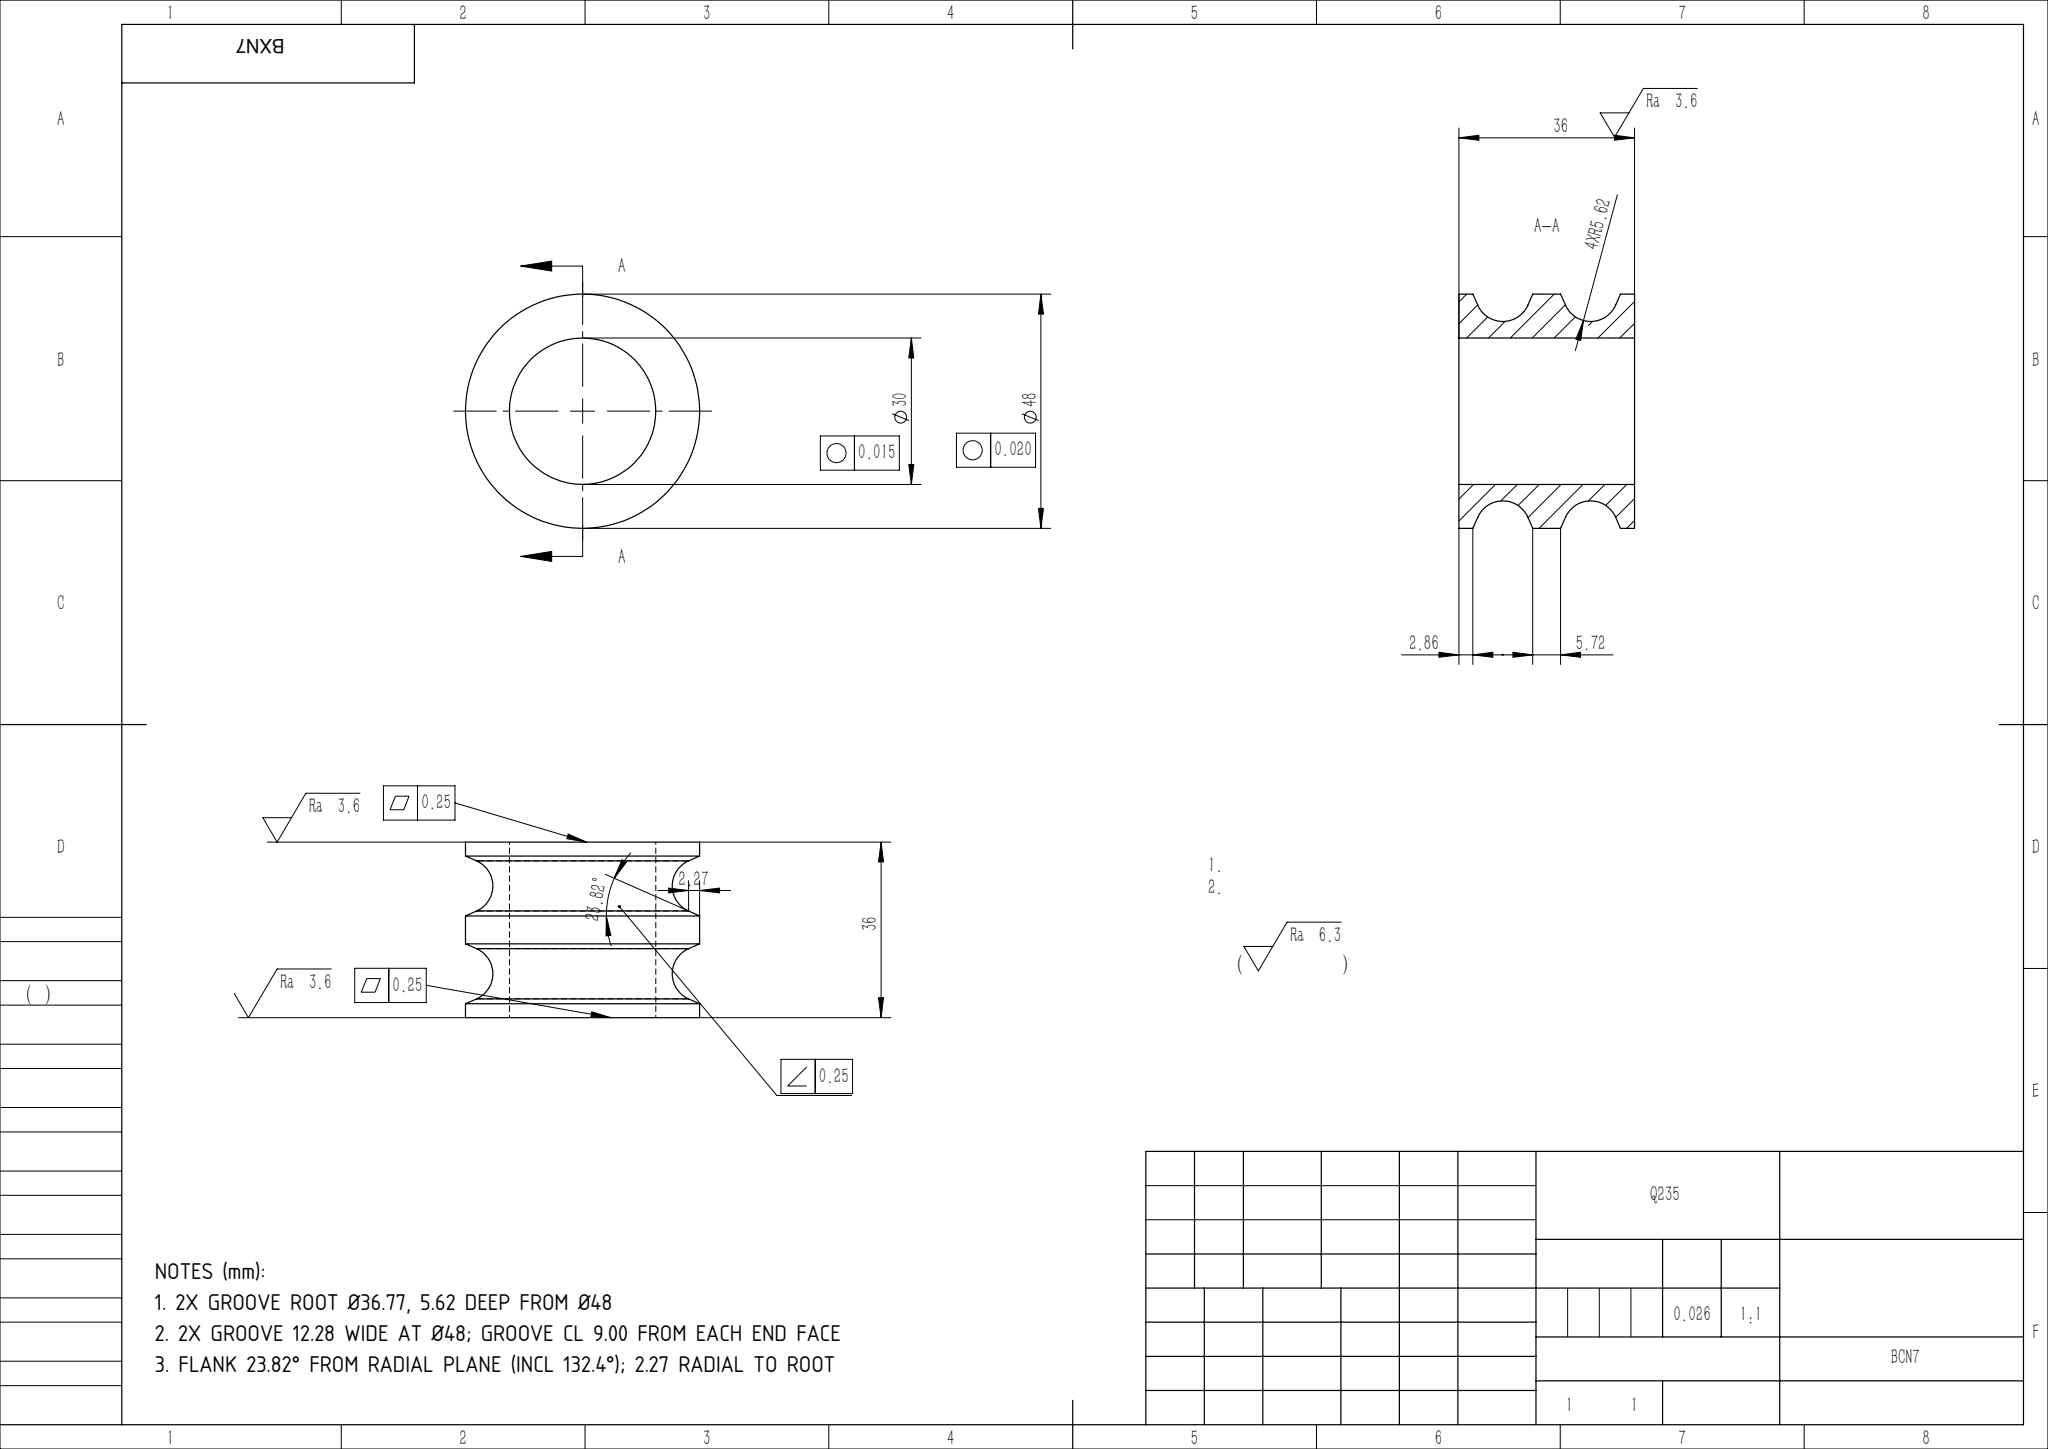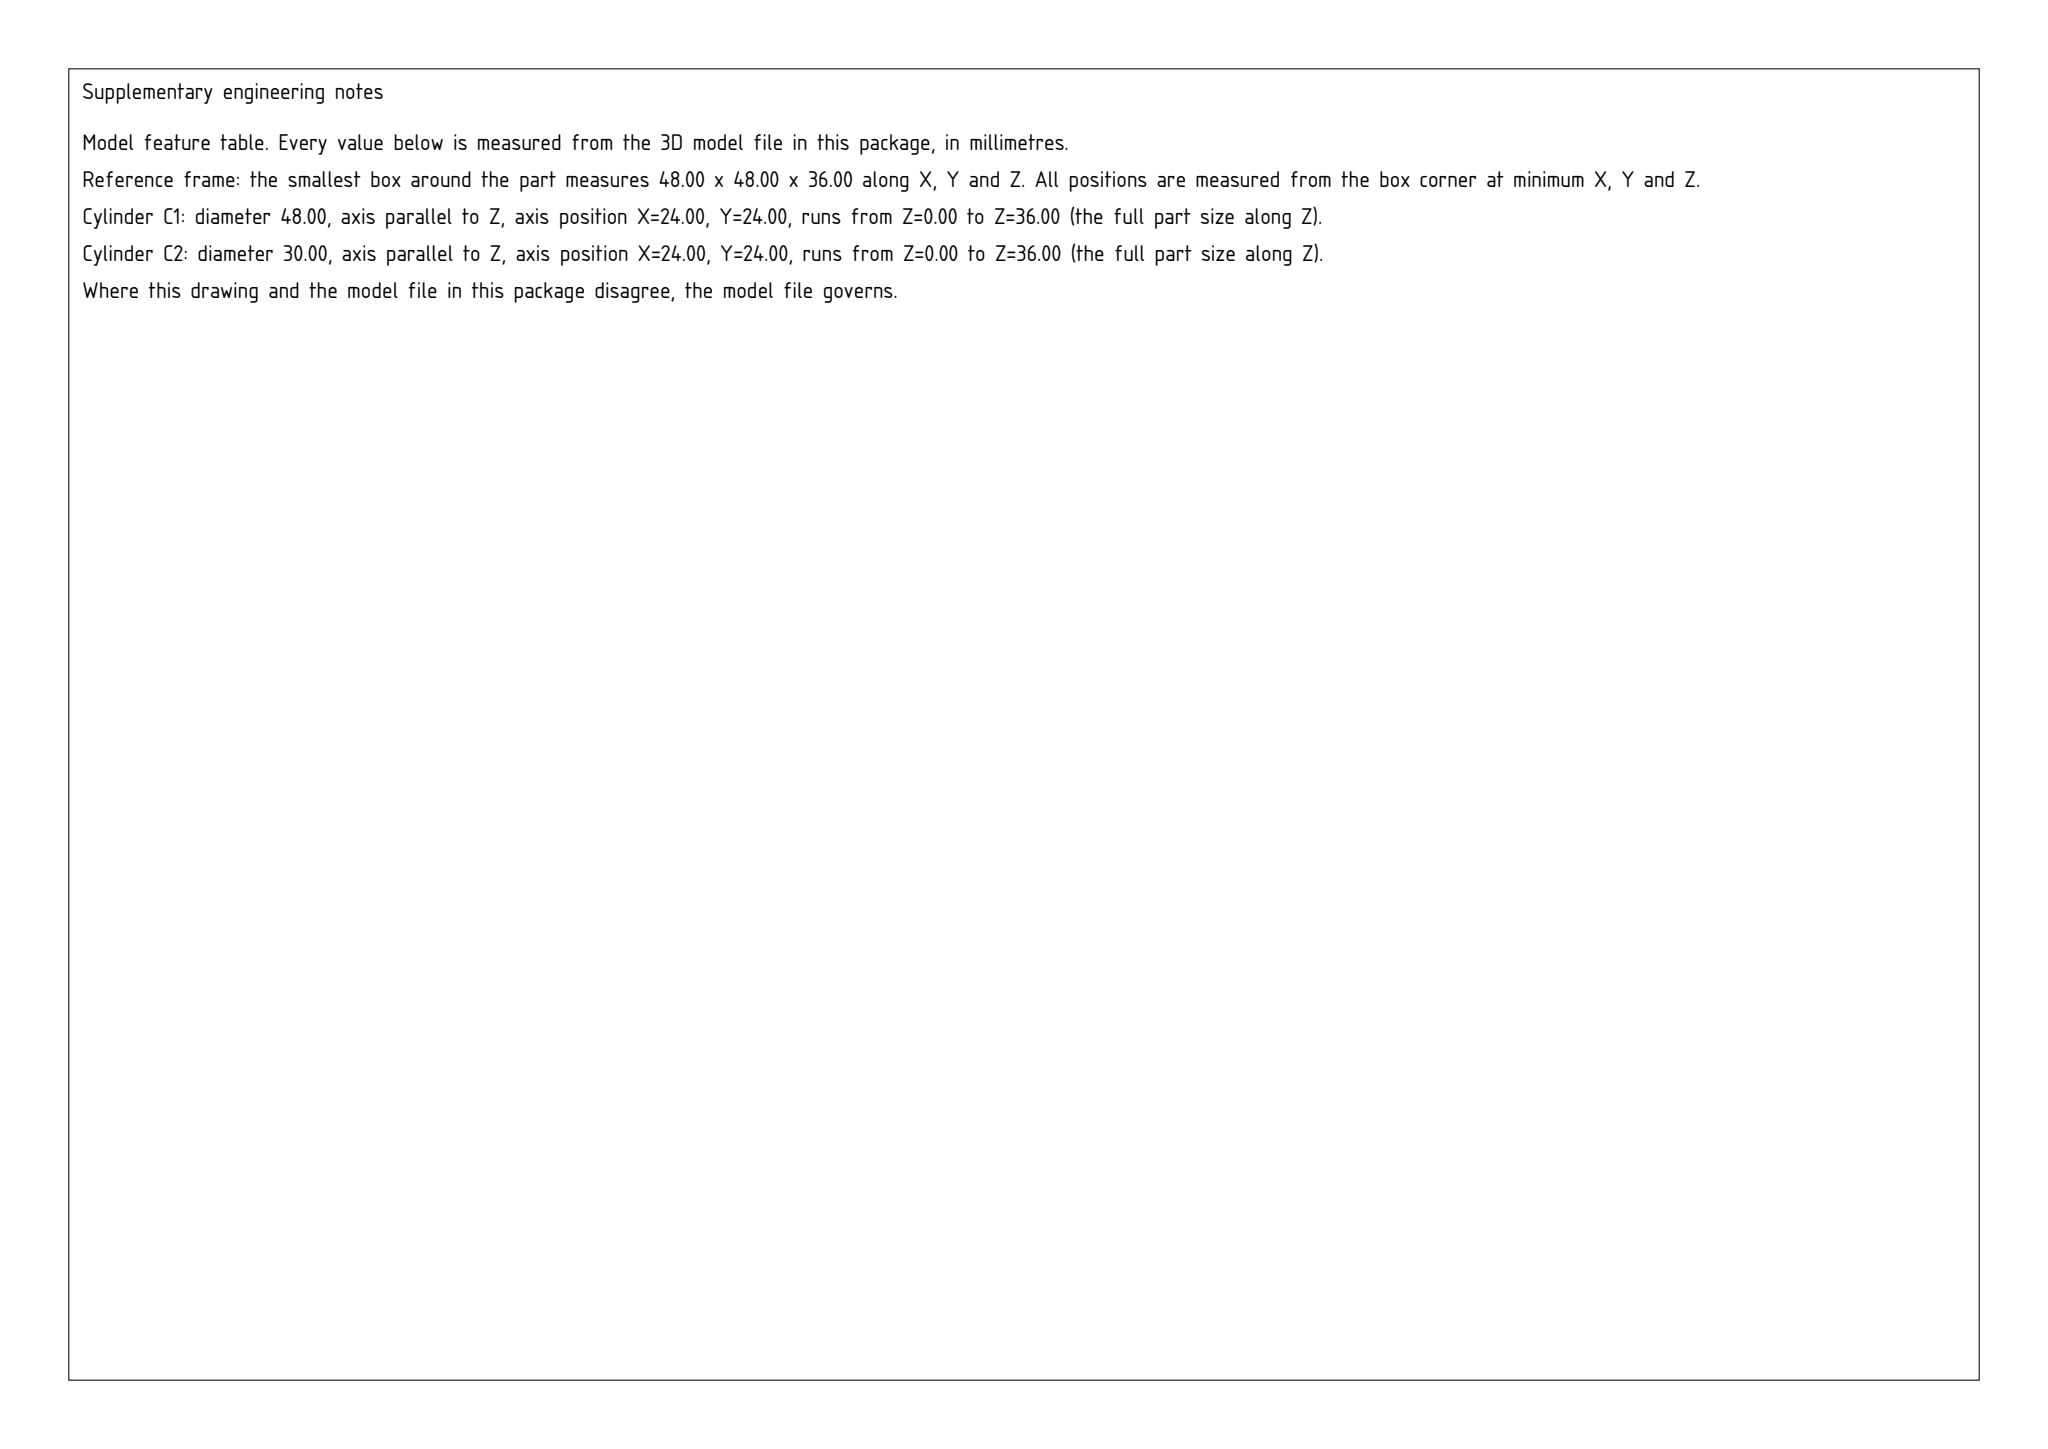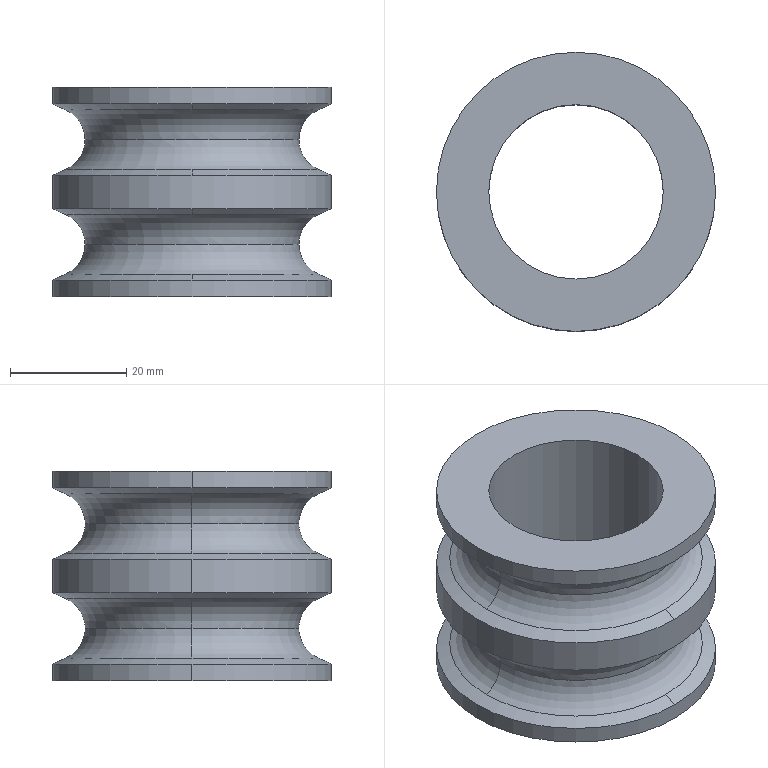Part | SolidWorks | mm | material Q235 | 1 solid | 26 faces | box 48 x 48 x 36 mm | volume 26002 mm3 | torus 8 | cylinder 8 | cone 8 | plane 2 | commonest cylinder face diameters 48 x6 30 x2
Drawing notes:
2X GROOVE ROOT Ø36.77, 5.62 DEEP FROM Ø48 | from the solid: cones incl angle 132.4 ref dia 48 tangent to R5.616 fillets -> root radius 18.384 (24-5.616), depth = R = 5.616
2X GROOVE 12.28 WIDE AT Ø48; GROOVE CL 9.00 FROM EACH END FACE | from the solid: 36 overall - (2.86+5.72+2.86) Ø48 lands = 24.56 / 2 grooves = 12.28 ea; CL = 2.86+6.14 = 9.00 from z=0 and z=36 faces
FLANK 23.82° FROM RADIAL PLANE (INCL 132.4°); 2.27 RADIAL TO ROOT | from the solid: cone included angle 132.4 deg about z = 23.8 deg from plane normal to axis; cone radial extent 20.652->18.384 = 2.268
STEP:
#1=CARTESIAN_POINT('',(-21.732,0.,-14.137));
#2=VERTEX_POINT('',#1);
#3=CARTESIAN_POINT('',(-18.384,0.,-9.));
#4=VERTEX_POINT('',#3);
#5=CARTESIAN_POINT('',(-24.,0.,-9.));
#6=DIRECTION('',(0.,-1.,0.));
#7=DIRECTION('',(0.,0.,-1.));
#8=AXIS2_PLACEMENT_3D('',#5,#6,#7);
#9=CIRCLE('',#8,5.616);
#10=EDGE_CURVE('',#2,#4,#9,.T.);
#11=ORIENTED_EDGE('',*,*,#10,.T.);
#12=CARTESIAN_POINT('',(18.384,0.,-9.));
#13=VERTEX_POINT('',#12);
#14=CARTESIAN_POINT('',(0.,0.,-9.));
#15=DIRECTION('',(0.,0.,-1.));
#16=DIRECTION('',(-1.,0.,0.));
#17=AXIS2_PLACEMENT_3D('',#14,#15,#16);
#18=CIRCLE('',#17,18.384);
#19=EDGE_CURVE('',#4,#13,#18,.T.);
#20=ORIENTED_EDGE('',*,*,#19,.T.);
#21=CARTESIAN_POINT('',(21.732,0.,-14.137));
#22=VERTEX_POINT('',#21);
#23=CARTESIAN_POINT('',(24.,0.,-9.));
#24=DIRECTION('',(-0.,1.,0.));
#25=DIRECTION('',(-1.,-0.,0.));
#26=AXIS2_PLACEMENT_3D('',#23,#24,#25);
#27=CIRCLE('',#26,5.616);
#28=EDGE_CURVE('',#22,#13,#27,.T.);
#29=ORIENTED_EDGE('',*,*,#28,.F.);
#30=CARTESIAN_POINT('',(0.,21.732,-14.137));
#31=VERTEX_POINT('',#30);
#32=CARTESIAN_POINT('',(0.,0.,-14.137));
#33=DIRECTION('',(0.,0.,-1.));
#34=DIRECTION('',(-1.,0.,0.));
#35=AXIS2_PLACEMENT_3D('',#32,#33,#34);
#36=CIRCLE('',#35,21.732);
#37=EDGE_CURVE('',#31,#22,#36,.T.);
#38=ORIENTED_EDGE('',*,*,#37,.F.);
#39=CARTESIAN_POINT('',(0.,0.,-14.137));
#40=DIRECTION('',(0.,0.,-1.));
#41=DIRECTION('',(-1.,0.,0.));
#42=AXIS2_PLACEMENT_3D('',#39,#40,#41);
#43=CIRCLE('',#42,21.732);
#44=EDGE_CURVE('',#2,#31,#43,.T.);
#45=ORIENTED_EDGE('',*,*,#44,.F.);
#46=EDGE_LOOP('',(#11,#20,#29,#38,#45));
#47=FACE_OUTER_BOUND('',#46,.T.);
#48=CARTESIAN_POINT('',(0.,0.,-9.));
#49=DIRECTION('',(0.,0.,-1.));
#50=DIRECTION('',(-1.,0.,0.));
#51=AXIS2_PLACEMENT_3D('',#48,#49,#50);
#52=TOROIDAL_SURFACE('',#51,24.,5.616);
#53=ADVANCED_FACE('',(#47),#52,.F.);
#54=CARTESIAN_POINT('',(21.732,0.,14.137));
#55=VERTEX_POINT('',#54);
#56=CARTESIAN_POINT('',(18.384,0.,9.));
#57=VERTEX_POINT('',#56);
#58=CARTESIAN_POINT('',(24.,0.,9.));
#59=DIRECTION('',(0.,-1.,0.));
#60=DIRECTION('',(0.,0.,-1.));
#61=AXIS2_PLACEMENT_3D('',#58,#59,#60);
#62=CIRCLE('',#61,5.616);
#63=EDGE_CURVE('',#55,#57,#62,.T.);
#64=ORIENTED_EDGE('',*,*,#63,.T.);
#65=CARTESIAN_POINT('',(-18.384,0.,9.));
#66=VERTEX_POINT('',#65);
#67=CARTESIAN_POINT('',(0.,0.,9.));
#68=DIRECTION('',(0.,0.,1.));
#69=DIRECTION('',(1.,0.,0.));
#70=AXIS2_PLACEMENT_3D('',#67,#68,#69);
#71=CIRCLE('',#70,18.384);
#72=EDGE_CURVE('',#57,#66,#71,.T.);
#73=ORIENTED_EDGE('',*,*,#72,.T.);
#74=CARTESIAN_POINT('',(-21.732,0.,14.137));
#75=VERTEX_POINT('',#74);
#76=CARTESIAN_POINT('',(-24.,0.,9.));
#77=DIRECTION('',(0.,1.,0.));
#78=DIRECTION('',(-1.,0.,0.));
#79=AXIS2_PLACEMENT_3D('',#76,#77,#78);
#80=CIRCLE('',#79,5.616);
#81=EDGE_CURVE('',#75,#66,#80,.T.);
#82=ORIENTED_EDGE('',*,*,#81,.F.);
#83=CARTESIAN_POINT('',(0.,21.732,14.137));
#84=VERTEX_POINT('',#83);
#85=CARTESIAN_POINT('',(0.,0.,14.137));
#86=DIRECTION('',(0.,0.,1.));
#87=DIRECTION('',(-1.,0.,0.));
#88=AXIS2_PLACEMENT_3D('',#85,#86,#87);
#89=CIRCLE('',#88,21.732);
#90=EDGE_CURVE('',#84,#75,#89,.T.);
#91=ORIENTED_EDGE('',*,*,#90,.F.);
#92=CARTESIAN_POINT('',(0.,0.,14.137));
#93=DIRECTION('',(0.,0.,1.));
#94=DIRECTION('',(-1.,0.,0.));
#95=AXIS2_PLACEMENT_3D('',#92,#93,#94);
#96=CIRCLE('',#95,21.732);
#97=EDGE_CURVE('',#55,#84,#96,.T.);
#98=ORIENTED_EDGE('',*,*,#97,.F.);
#99=EDGE_LOOP('',(#64,#73,#82,#91,#98));
#100=FACE_OUTER_BOUND('',#99,.T.);
#101=CARTESIAN_POINT('',(0.,0.,9.));
#102=DIRECTION('',(0.,0.,1.));
#103=DIRECTION('',(1.,0.,0.));
#104=AXIS2_PLACEMENT_3D('',#101,#102,#103);
#105=TOROIDAL_SURFACE('',#104,24.,5.616);
#106=ADVANCED_FACE('',(#100),#105,.F.);
#107=ORIENTED_EDGE('',*,*,#81,.T.);
#108=CARTESIAN_POINT('',(0.,0.,9.));
#109=DIRECTION('',(0.,0.,1.));
#110=DIRECTION('',(1.,0.,0.));
#111=AXIS2_PLACEMENT_3D('',#108,#109,#110);
#112=CIRCLE('',#111,18.384);
#113=EDGE_CURVE('',#66,#57,#112,.T.);
#114=ORIENTED_EDGE('',*,*,#113,.T.);
#115=ORIENTED_EDGE('',*,*,#63,.F.);
#116=CARTESIAN_POINT('',(0.,-21.732,14.137));
#117=VERTEX_POINT('',#116);
#118=CARTESIAN_POINT('',(0.,0.,14.137));
#119=DIRECTION('',(0.,0.,1.));
#120=DIRECTION('',(-1.,0.,0.));
#121=AXIS2_PLACEMENT_3D('',#118,#119,#120);
#122=CIRCLE('',#121,21.732);
#123=EDGE_CURVE('',#117,#55,#122,.T.);
#124=ORIENTED_EDGE('',*,*,#123,.F.);
#125=CARTESIAN_POINT('',(0.,0.,14.137));
#126=DIRECTION('',(0.,0.,1.));
#127=DIRECTION('',(-1.,0.,0.));
#128=AXIS2_PLACEMENT_3D('',#125,#126,#127);
#129=CIRCLE('',#128,21.732);
#130=EDGE_CURVE('',#75,#117,#129,.T.);
#131=ORIENTED_EDGE('',*,*,#130,.F.);
#132=EDGE_LOOP('',(#107,#114,#115,#124,#131));
#133=FACE_OUTER_BOUND('',#132,.T.);
#134=CARTESIAN_POINT('',(0.,0.,9.));
#135=DIRECTION('',(0.,0.,1.));
#136=DIRECTION('',(1.,0.,0.));
#137=AXIS2_PLACEMENT_3D('',#134,#135,#136);
#138=TOROIDAL_SURFACE('',#137,24.,5.616);
#139=ADVANCED_FACE('',(#133),#138,.F.);
#140=ORIENTED_EDGE('',*,*,#28,.T.);
#141=CARTESIAN_POINT('',(0.,0.,-9.));
#142=DIRECTION('',(0.,0.,-1.));
#143=DIRECTION('',(-1.,0.,0.));
#144=AXIS2_PLACEMENT_3D('',#141,#142,#143);
#145=CIRCLE('',#144,18.384);
#146=EDGE_CURVE('',#13,#4,#145,.T.);
#147=ORIENTED_EDGE('',*,*,#146,.T.);
#148=ORIENTED_EDGE('',*,*,#10,.F.);
#149=CARTESIAN_POINT('',(0.,-21.732,-14.137));
#150=VERTEX_POINT('',#149);
#151=CARTESIAN_POINT('',(0.,0.,-14.137));
#152=DIRECTION('',(0.,0.,-1.));
#153=DIRECTION('',(-1.,0.,0.));
#154=AXIS2_PLACEMENT_3D('',#151,#152,#153);
#155=CIRCLE('',#154,21.732);
#156=EDGE_CURVE('',#150,#2,#155,.T.);
#157=ORIENTED_EDGE('',*,*,#156,.F.);
#158=CARTESIAN_POINT('',(0.,0.,-14.137));
#159=DIRECTION('',(0.,0.,-1.));
#160=DIRECTION('',(-1.,0.,0.));
#161=AXIS2_PLACEMENT_3D('',#158,#159,#160);
#162=CIRCLE('',#161,21.732);
#163=EDGE_CURVE('',#22,#150,#162,.T.);
#164=ORIENTED_EDGE('',*,*,#163,.F.);
#165=EDGE_LOOP('',(#140,#147,#148,#157,#164));
#166=FACE_OUTER_BOUND('',#165,.T.);
#167=CARTESIAN_POINT('',(0.,0.,-9.));
#168=DIRECTION('',(0.,0.,-1.));
#169=DIRECTION('',(-1.,0.,0.));
#170=AXIS2_PLACEMENT_3D('',#167,#168,#169);
#171=TOROIDAL_SURFACE('',#170,24.,5.616);
#172=ADVANCED_FACE('',(#166),#171,.F.);
#173=CARTESIAN_POINT('',(-15.,0.,-18.));
#174=VERTEX_POINT('',#173);
#175=CARTESIAN_POINT('',(15.,0.,-18.));
#176=VERTEX_POINT('',#175);
#177=CARTESIAN_POINT('',(0.,0.,-18.));
#178=DIRECTION('',(0.,0.,1.));
#179=DIRECTION('',(1.,0.,0.));
#180=AXIS2_PLACEMENT_3D('',#177,#178,#179);
#181=CIRCLE('',#180,15.);
#182=EDGE_CURVE('',#174,#176,#181,.T.);
#183=ORIENTED_EDGE('',*,*,#182,.F.);
#184=CARTESIAN_POINT('',(-15.,0.,18.));
#185=VERTEX_POINT('',#184);
#186=CARTESIAN_POINT('',(-15.,0.,-18.));
#187=DIRECTION('',(0.,0.,1.));
#188=VECTOR('',#187,1000.);
#189=LINE('',#186,#188);
#190=EDGE_CURVE('',#174,#185,#189,.T.);
#191=ORIENTED_EDGE('',*,*,#190,.T.);
#192=CARTESIAN_POINT('',(15.,0.,18.));
#193=VERTEX_POINT('',#192);
#194=CARTESIAN_POINT('',(0.,0.,18.));
#195=DIRECTION('',(0.,0.,-1.));
#196=DIRECTION('',(1.,0.,0.));
#197=AXIS2_PLACEMENT_3D('',#194,#195,#196);
#198=CIRCLE('',#197,15.);
#199=EDGE_CURVE('',#193,#185,#198,.T.);
#200=ORIENTED_EDGE('',*,*,#199,.F.);
#201=CARTESIAN_POINT('',(15.,0.,-18.));
#202=DIRECTION('',(0.,0.,1.));
#203=VECTOR('',#202,1000.);
#204=LINE('',#201,#203);
#205=EDGE_CURVE('',#176,#193,#204,.T.);
#206=ORIENTED_EDGE('',*,*,#205,.F.);
#207=EDGE_LOOP('',(#183,#191,#200,#206));
#208=FACE_OUTER_BOUND('',#207,.T.);
#209=CARTESIAN_POINT('',(0.,0.,-18.));
#210=DIRECTION('',(0.,0.,1.));
#211=DIRECTION('',(1.,0.,0.));
#212=AXIS2_PLACEMENT_3D('',#209,#210,#211);
#213=CYLINDRICAL_SURFACE('',#212,15.);
#214=ADVANCED_FACE('',(#208),#213,.F.);
#215=CARTESIAN_POINT('',(24.,0.,-18.));
#216=VERTEX_POINT('',#215);
#217=CARTESIAN_POINT('',(-24.,0.,-18.));
#218=VERTEX_POINT('',#217);
#219=CARTESIAN_POINT('',(0.,0.,-18.));
#220=DIRECTION('',(0.,0.,1.));
#221=DIRECTION('',(1.,0.,0.));
#222=AXIS2_PLACEMENT_3D('',#219,#220,#221);
#223=CIRCLE('',#222,24.);
#224=EDGE_CURVE('',#216,#218,#223,.T.);
#225=ORIENTED_EDGE('',*,*,#224,.T.);
#226=CARTESIAN_POINT('',(-24.,0.,-15.138));
#227=VERTEX_POINT('',#226);
#228=CARTESIAN_POINT('',(-24.,0.,-18.));
#229=DIRECTION('',(0.,0.,1.));
#230=VECTOR('',#229,1000.);
#231=LINE('',#228,#230);
#232=EDGE_CURVE('',#218,#227,#231,.T.);
#233=ORIENTED_EDGE('',*,*,#232,.T.);
#234=CARTESIAN_POINT('',(0.,24.,-15.138));
#235=VERTEX_POINT('',#234);
#236=CARTESIAN_POINT('',(0.,0.,-15.138));
#237=DIRECTION('',(0.,0.,-1.));
#238=DIRECTION('',(1.,0.,0.));
#239=AXIS2_PLACEMENT_3D('',#236,#237,#238);
#240=CIRCLE('',#239,24.);
#241=EDGE_CURVE('',#227,#235,#240,.T.);
#242=ORIENTED_EDGE('',*,*,#241,.T.);
#243=CARTESIAN_POINT('',(24.,0.,-15.138));
#244=VERTEX_POINT('',#243);
#245=CARTESIAN_POINT('',(0.,0.,-15.138));
#246=DIRECTION('',(0.,0.,-1.));
#247=DIRECTION('',(1.,0.,0.));
#248=AXIS2_PLACEMENT_3D('',#245,#246,#247);
#249=CIRCLE('',#248,24.);
#250=EDGE_CURVE('',#235,#244,#249,.T.);
#251=ORIENTED_EDGE('',*,*,#250,.T.);
#252=CARTESIAN_POINT('',(24.,0.,-18.));
#253=DIRECTION('',(0.,0.,1.));
#254=VECTOR('',#253,1000.);
#255=LINE('',#252,#254);
#256=EDGE_CURVE('',#216,#244,#255,.T.);
#257=ORIENTED_EDGE('',*,*,#256,.F.);
#258=EDGE_LOOP('',(#225,#233,#242,#251,#257));
#259=FACE_OUTER_BOUND('',#258,.T.);
#260=CARTESIAN_POINT('',(0.,0.,-18.));
#261=DIRECTION('',(0.,0.,1.));
#262=DIRECTION('',(1.,0.,0.));
#263=AXIS2_PLACEMENT_3D('',#260,#261,#262);
#264=CYLINDRICAL_SURFACE('',#263,24.);
#265=ADVANCED_FACE('',(#259),#264,.T.);
#266=CARTESIAN_POINT('',(-24.,0.,18.));
#267=VERTEX_POINT('',#266);
#268=CARTESIAN_POINT('',(24.,0.,18.));
#269=VERTEX_POINT('',#268);
#270=CARTESIAN_POINT('',(0.,0.,18.));
#271=DIRECTION('',(0.,0.,-1.));
#272=DIRECTION('',(-1.,0.,0.));
#273=AXIS2_PLACEMENT_3D('',#270,#271,#272);
#274=CIRCLE('',#273,24.);
#275=EDGE_CURVE('',#267,#269,#274,.T.);
#276=ORIENTED_EDGE('',*,*,#275,.T.);
#277=CARTESIAN_POINT('',(24.,0.,15.138));
#278=VERTEX_POINT('',#277);
#279=CARTESIAN_POINT('',(24.,0.,18.));
#280=DIRECTION('',(0.,0.,-1.));
#281=VECTOR('',#280,1000.);
#282=LINE('',#279,#281);
#283=EDGE_CURVE('',#269,#278,#282,.T.);
#284=ORIENTED_EDGE('',*,*,#283,.T.);
#285=CARTESIAN_POINT('',(0.,24.,15.138));
#286=VERTEX_POINT('',#285);
#287=CARTESIAN_POINT('',(0.,0.,15.138));
#288=DIRECTION('',(0.,0.,1.));
#289=DIRECTION('',(-1.,0.,0.));
#290=AXIS2_PLACEMENT_3D('',#287,#288,#289);
#291=CIRCLE('',#290,24.);
#292=EDGE_CURVE('',#278,#286,#291,.T.);
#293=ORIENTED_EDGE('',*,*,#292,.T.);
#294=CARTESIAN_POINT('',(-24.,0.,15.138));
#295=VERTEX_POINT('',#294);
#296=CARTESIAN_POINT('',(0.,0.,15.138));
#297=DIRECTION('',(0.,0.,1.));
#298=DIRECTION('',(-1.,0.,0.));
#299=AXIS2_PLACEMENT_3D('',#296,#297,#298);
#300=CIRCLE('',#299,24.);
#301=EDGE_CURVE('',#286,#295,#300,.T.);
#302=ORIENTED_EDGE('',*,*,#301,.T.);
#303=CARTESIAN_POINT('',(-24.,0.,18.));
#304=DIRECTION('',(0.,0.,-1.));
#305=VECTOR('',#304,1000.);
#306=LINE('',#303,#305);
#307=EDGE_CURVE('',#267,#295,#306,.T.);
#308=ORIENTED_EDGE('',*,*,#307,.F.);
#309=EDGE_LOOP('',(#276,#284,#293,#302,#308));
#310=FACE_OUTER_BOUND('',#309,.T.);
#311=CARTESIAN_POINT('',(0.,0.,18.));
#312=DIRECTION('',(0.,0.,-1.));
#313=DIRECTION('',(-1.,0.,0.));
#314=AXIS2_PLACEMENT_3D('',#311,#312,#313);
#315=CYLINDRICAL_SURFACE('',#314,24.);
#316=ADVANCED_FACE('',(#310),#315,.T.);
#317=ORIENTED_EDGE('',*,*,#163,.T.);
#318=CARTESIAN_POINT('',(0.,-24.,-15.138));
#319=VERTEX_POINT('',#318);
#320=CARTESIAN_POINT('',(0.,-24.,-15.138));
#321=DIRECTION('',(0.,-0.9148,-0.4038));
#322=VECTOR('',#321,1000.);
#323=LINE('',#320,#322);
#324=EDGE_CURVE('',#150,#319,#323,.T.);
#325=ORIENTED_EDGE('',*,*,#324,.T.);
#326=CARTESIAN_POINT('',(0.,0.,-15.138));
#327=DIRECTION('',(0.,0.,-1.));
#328=DIRECTION('',(1.,0.,0.));
#329=AXIS2_PLACEMENT_3D('',#326,#327,#328);
#330=CIRCLE('',#329,24.);
#331=EDGE_CURVE('',#244,#319,#330,.T.);
#332=ORIENTED_EDGE('',*,*,#331,.F.);
#333=ORIENTED_EDGE('',*,*,#250,.F.);
#334=CARTESIAN_POINT('',(0.,24.,-15.138));
#335=DIRECTION('',(0.,0.9148,-0.4038));
#336=VECTOR('',#335,1000.);
#337=LINE('',#334,#336);
#338=EDGE_CURVE('',#31,#235,#337,.T.);
#339=ORIENTED_EDGE('',*,*,#338,.F.);
#340=ORIENTED_EDGE('',*,*,#37,.T.);
#341=EDGE_LOOP('',(#317,#325,#332,#333,#339,#340));
#342=FACE_OUTER_BOUND('',#341,.T.);
#343=CARTESIAN_POINT('',(0.,0.,-15.138));
#344=DIRECTION('',(0.,0.,-1.));
#345=DIRECTION('',(0.,1.,0.));
#346=AXIS2_PLACEMENT_3D('',#343,#344,#345);
#347=CONICAL_SURFACE('',#346,24.,1.155);
#348=ADVANCED_FACE('',(#342),#347,.T.);
#349=ORIENTED_EDGE('',*,*,#97,.T.);
#350=CARTESIAN_POINT('',(0.,24.,15.138));
#351=DIRECTION('',(0.,0.9148,0.4038));
#352=VECTOR('',#351,1000.);
#353=LINE('',#350,#352);
#354=EDGE_CURVE('',#84,#286,#353,.T.);
#355=ORIENTED_EDGE('',*,*,#354,.T.);
#356=ORIENTED_EDGE('',*,*,#292,.F.);
#357=CARTESIAN_POINT('',(0.,-24.,15.138));
#358=VERTEX_POINT('',#357);
#359=CARTESIAN_POINT('',(0.,0.,15.138));
#360=DIRECTION('',(0.,0.,1.));
#361=DIRECTION('',(-1.,0.,0.));
#362=AXIS2_PLACEMENT_3D('',#359,#360,#361);
#363=CIRCLE('',#362,24.);
#364=EDGE_CURVE('',#358,#278,#363,.T.);
#365=ORIENTED_EDGE('',*,*,#364,.F.);
#366=CARTESIAN_POINT('',(0.,-24.,15.138));
#367=DIRECTION('',(0.,-0.9148,0.4038));
#368=VECTOR('',#367,1000.);
#369=LINE('',#366,#368);
#370=EDGE_CURVE('',#117,#358,#369,.T.);
#371=ORIENTED_EDGE('',*,*,#370,.F.);
#372=ORIENTED_EDGE('',*,*,#123,.T.);
#373=EDGE_LOOP('',(#349,#355,#356,#365,#371,#372));
#374=FACE_OUTER_BOUND('',#373,.T.);
#375=CARTESIAN_POINT('',(0.,0.,15.138));
#376=DIRECTION('',(0.,-0.,1.));
#377=DIRECTION('',(0.,-1.,-0.));
#378=AXIS2_PLACEMENT_3D('',#375,#376,#377);
#379=CONICAL_SURFACE('',#378,24.,1.155);
#380=ADVANCED_FACE('',(#374),#379,.T.);
#381=ORIENTED_EDGE('',*,*,#146,.F.);
#382=CARTESIAN_POINT('',(21.732,0.,-3.863));
#383=VERTEX_POINT('',#382);
#384=CARTESIAN_POINT('',(24.,0.,-9.));
#385=DIRECTION('',(-0.,1.,0.));
#386=DIRECTION('',(-1.,-0.,0.));
#387=AXIS2_PLACEMENT_3D('',#384,#385,#386);
#388=CIRCLE('',#387,5.616);
#389=EDGE_CURVE('',#13,#383,#388,.T.);
#390=ORIENTED_EDGE('',*,*,#389,.T.);
#391=CARTESIAN_POINT('',(-0.,-21.732,-3.863));
#392=VERTEX_POINT('',#391);
#393=CARTESIAN_POINT('',(0.,0.,-3.863));
#394=DIRECTION('',(0.,0.,1.));
#395=DIRECTION('',(1.,0.,0.));
#396=AXIS2_PLACEMENT_3D('',#393,#394,#395);
#397=CIRCLE('',#396,21.732);
#398=EDGE_CURVE('',#392,#383,#397,.T.);
#399=ORIENTED_EDGE('',*,*,#398,.F.);
#400=CARTESIAN_POINT('',(-21.732,0.,-3.863));
#401=VERTEX_POINT('',#400);
#402=CARTESIAN_POINT('',(0.,0.,-3.863));
#403=DIRECTION('',(0.,0.,1.));
#404=DIRECTION('',(1.,0.,0.));
#405=AXIS2_PLACEMENT_3D('',#402,#403,#404);
#406=CIRCLE('',#405,21.732);
#407=EDGE_CURVE('',#401,#392,#406,.T.);
#408=ORIENTED_EDGE('',*,*,#407,.F.);
#409=CARTESIAN_POINT('',(-24.,0.,-9.));
#410=DIRECTION('',(0.,-1.,0.));
#411=DIRECTION('',(0.,0.,-1.));
#412=AXIS2_PLACEMENT_3D('',#409,#410,#411);
#413=CIRCLE('',#412,5.616);
#414=EDGE_CURVE('',#4,#401,#413,.T.);
#415=ORIENTED_EDGE('',*,*,#414,.F.);
#416=EDGE_LOOP('',(#381,#390,#399,#408,#415));
#417=FACE_OUTER_BOUND('',#416,.T.);
#418=CARTESIAN_POINT('',(0.,0.,-9.));
#419=DIRECTION('',(0.,0.,-1.));
#420=DIRECTION('',(-1.,0.,0.));
#421=AXIS2_PLACEMENT_3D('',#418,#419,#420);
#422=TOROIDAL_SURFACE('',#421,24.,5.616);
#423=ADVANCED_FACE('',(#417),#422,.F.);
#424=ORIENTED_EDGE('',*,*,#113,.F.);
#425=CARTESIAN_POINT('',(-21.732,0.,3.863));
#426=VERTEX_POINT('',#425);
#427=CARTESIAN_POINT('',(-24.,0.,9.));
#428=DIRECTION('',(0.,1.,0.));
#429=DIRECTION('',(-1.,0.,0.));
#430=AXIS2_PLACEMENT_3D('',#427,#428,#429);
#431=CIRCLE('',#430,5.616);
#432=EDGE_CURVE('',#66,#426,#431,.T.);
#433=ORIENTED_EDGE('',*,*,#432,.T.);
#434=CARTESIAN_POINT('',(0.,-21.732,3.863));
#435=VERTEX_POINT('',#434);
#436=CARTESIAN_POINT('',(0.,0.,3.863));
#437=DIRECTION('',(0.,0.,-1.));
#438=DIRECTION('',(-1.,0.,0.));
#439=AXIS2_PLACEMENT_3D('',#436,#437,#438);
#440=CIRCLE('',#439,21.732);
#441=EDGE_CURVE('',#435,#426,#440,.T.);
#442=ORIENTED_EDGE('',*,*,#441,.F.);
#443=CARTESIAN_POINT('',(21.732,0.,3.863));
#444=VERTEX_POINT('',#443);
#445=CARTESIAN_POINT('',(0.,0.,3.863));
#446=DIRECTION('',(0.,0.,-1.));
#447=DIRECTION('',(-1.,0.,0.));
#448=AXIS2_PLACEMENT_3D('',#445,#446,#447);
#449=CIRCLE('',#448,21.732);
#450=EDGE_CURVE('',#444,#435,#449,.T.);
#451=ORIENTED_EDGE('',*,*,#450,.F.);
#452=CARTESIAN_POINT('',(24.,0.,9.));
#453=DIRECTION('',(0.,-1.,0.));
#454=DIRECTION('',(0.,0.,-1.));
#455=AXIS2_PLACEMENT_3D('',#452,#453,#454);
#456=CIRCLE('',#455,5.616);
#457=EDGE_CURVE('',#57,#444,#456,.T.);
#458=ORIENTED_EDGE('',*,*,#457,.F.);
#459=EDGE_LOOP('',(#424,#433,#442,#451,#458));
#460=FACE_OUTER_BOUND('',#459,.T.);
#461=CARTESIAN_POINT('',(0.,0.,9.));
#462=DIRECTION('',(0.,0.,1.));
#463=DIRECTION('',(1.,0.,0.));
#464=AXIS2_PLACEMENT_3D('',#461,#462,#463);
#465=TOROIDAL_SURFACE('',#464,24.,5.616);
#466=ADVANCED_FACE('',(#460),#465,.F.);
#467=ORIENTED_EDGE('',*,*,#398,.T.);
#468=CARTESIAN_POINT('',(0.,21.732,-3.863));
#469=VERTEX_POINT('',#468);
#470=CARTESIAN_POINT('',(0.,0.,-3.863));
#471=DIRECTION('',(0.,0.,1.));
#472=DIRECTION('',(1.,0.,0.));
#473=AXIS2_PLACEMENT_3D('',#470,#471,#472);
#474=CIRCLE('',#473,21.732);
#475=EDGE_CURVE('',#383,#469,#474,.T.);
#476=ORIENTED_EDGE('',*,*,#475,.T.);
#477=CARTESIAN_POINT('',(0.,24.,-2.862));
#478=VERTEX_POINT('',#477);
#479=CARTESIAN_POINT('',(0.,24.,-2.862));
#480=DIRECTION('',(0.,0.9148,0.4038));
#481=VECTOR('',#480,1000.);
#482=LINE('',#479,#481);
#483=EDGE_CURVE('',#469,#478,#482,.T.);
#484=ORIENTED_EDGE('',*,*,#483,.T.);
#485=CARTESIAN_POINT('',(24.,-0.,-2.862));
#486=VERTEX_POINT('',#485);
#487=CARTESIAN_POINT('',(0.,0.,-2.862));
#488=DIRECTION('',(0.,0.,-1.));
#489=DIRECTION('',(0.,-1.,-0.));
#490=AXIS2_PLACEMENT_3D('',#487,#488,#489);
#491=CIRCLE('',#490,24.);
#492=EDGE_CURVE('',#478,#486,#491,.T.);
#493=ORIENTED_EDGE('',*,*,#492,.T.);
#494=CARTESIAN_POINT('',(0.,-24.,-2.862));
#495=VERTEX_POINT('',#494);
#496=CARTESIAN_POINT('',(0.,0.,-2.862));
#497=DIRECTION('',(0.,0.,-1.));
#498=DIRECTION('',(0.,-1.,-0.));
#499=AXIS2_PLACEMENT_3D('',#496,#497,#498);
#500=CIRCLE('',#499,24.);
#501=EDGE_CURVE('',#486,#495,#500,.T.);
#502=ORIENTED_EDGE('',*,*,#501,.T.);
#503=CARTESIAN_POINT('',(0.,-24.,-2.862));
#504=DIRECTION('',(0.,-0.9148,0.4038));
#505=VECTOR('',#504,1000.);
#506=LINE('',#503,#505);
#507=EDGE_CURVE('',#392,#495,#506,.T.);
#508=ORIENTED_EDGE('',*,*,#507,.F.);
#509=EDGE_LOOP('',(#467,#476,#484,#493,#502,#508));
#510=FACE_OUTER_BOUND('',#509,.T.);
#511=CARTESIAN_POINT('',(0.,-0.,-2.862));
#512=DIRECTION('',(0.,-0.,1.));
#513=DIRECTION('',(0.,-1.,-0.));
#514=AXIS2_PLACEMENT_3D('',#511,#512,#513);
#515=CONICAL_SURFACE('',#514,24.,1.155);
#516=ADVANCED_FACE('',(#510),#515,.T.);
#517=CARTESIAN_POINT('',(0.,21.732,3.863));
#518=VERTEX_POINT('',#517);
#519=CARTESIAN_POINT('',(0.,0.,3.863));
#520=DIRECTION('',(0.,0.,-1.));
#521=DIRECTION('',(-1.,0.,0.));
#522=AXIS2_PLACEMENT_3D('',#519,#520,#521);
#523=CIRCLE('',#522,21.732);
#524=EDGE_CURVE('',#518,#444,#523,.T.);
#525=ORIENTED_EDGE('',*,*,#524,.T.);
#526=ORIENTED_EDGE('',*,*,#450,.T.);
#527=CARTESIAN_POINT('',(0.,-24.,2.862));
#528=VERTEX_POINT('',#527);
#529=CARTESIAN_POINT('',(0.,-24.,2.862));
#530=DIRECTION('',(0.,-0.9148,-0.4038));
#531=VECTOR('',#530,1000.);
#532=LINE('',#529,#531);
#533=EDGE_CURVE('',#435,#528,#532,.T.);
#534=ORIENTED_EDGE('',*,*,#533,.T.);
#535=CARTESIAN_POINT('',(24.,-0.,2.862));
#536=VERTEX_POINT('',#535);
#537=CARTESIAN_POINT('',(0.,0.,2.862));
#538=DIRECTION('',(0.,0.,1.));
#539=DIRECTION('',(0.,-1.,0.));
#540=AXIS2_PLACEMENT_3D('',#537,#538,#539);
#541=CIRCLE('',#540,24.);
#542=EDGE_CURVE('',#528,#536,#541,.T.);
#543=ORIENTED_EDGE('',*,*,#542,.T.);
#544=CARTESIAN_POINT('',(-0.,24.,2.862));
#545=VERTEX_POINT('',#544);
#546=CARTESIAN_POINT('',(0.,0.,2.862));
#547=DIRECTION('',(0.,0.,1.));
#548=DIRECTION('',(0.,-1.,0.));
#549=AXIS2_PLACEMENT_3D('',#546,#547,#548);
#550=CIRCLE('',#549,24.);
#551=EDGE_CURVE('',#536,#545,#550,.T.);
#552=ORIENTED_EDGE('',*,*,#551,.T.);
#553=CARTESIAN_POINT('',(-0.,24.,2.862));
#554=DIRECTION('',(-0.,0.9148,-0.4038));
#555=VECTOR('',#554,1000.);
#556=LINE('',#553,#555);
#557=EDGE_CURVE('',#518,#545,#556,.T.);
#558=ORIENTED_EDGE('',*,*,#557,.F.);
#559=EDGE_LOOP('',(#525,#526,#534,#543,#552,#558));
#560=FACE_OUTER_BOUND('',#559,.T.);
#561=CARTESIAN_POINT('',(-0.,-0.,2.862));
#562=DIRECTION('',(-0.,-0.,-1.));
#563=DIRECTION('',(0.,1.,-0.));
#564=AXIS2_PLACEMENT_3D('',#561,#562,#563);
#565=CONICAL_SURFACE('',#564,24.,1.155);
#566=ADVANCED_FACE('',(#560),#565,.T.);
#567=CARTESIAN_POINT('',(-24.,0.,-2.862));
#568=VERTEX_POINT('',#567);
#569=CARTESIAN_POINT('',(0.,0.,-2.862));
#570=DIRECTION('',(0.,0.,-1.));
#571=DIRECTION('',(0.,-1.,-0.));
#572=AXIS2_PLACEMENT_3D('',#569,#570,#571);
#573=CIRCLE('',#572,24.);
#574=EDGE_CURVE('',#568,#478,#573,.T.);
#575=ORIENTED_EDGE('',*,*,#574,.F.);
#576=CARTESIAN_POINT('',(-24.,0.,2.862));
#577=VERTEX_POINT('',#576);
#578=CARTESIAN_POINT('',(-24.,0.,-18.));
#579=DIRECTION('',(0.,0.,1.));
#580=VECTOR('',#579,1000.);
#581=LINE('',#578,#580);
#582=EDGE_CURVE('',#568,#577,#581,.T.);
#583=ORIENTED_EDGE('',*,*,#582,.T.);
#584=CARTESIAN_POINT('',(0.,0.,2.862));
#585=DIRECTION('',(0.,0.,1.));
#586=DIRECTION('',(0.,-1.,0.));
#587=AXIS2_PLACEMENT_3D('',#584,#585,#586);
#588=CIRCLE('',#587,24.);
#589=EDGE_CURVE('',#545,#577,#588,.T.);
#590=ORIENTED_EDGE('',*,*,#589,.F.);
#591=ORIENTED_EDGE('',*,*,#551,.F.);
#592=CARTESIAN_POINT('',(24.,0.,-18.));
#593=DIRECTION('',(0.,0.,1.));
#594=VECTOR('',#593,1000.);
#595=LINE('',#592,#594);
#596=EDGE_CURVE('',#486,#536,#595,.T.);
#597=ORIENTED_EDGE('',*,*,#596,.F.);
#598=ORIENTED_EDGE('',*,*,#492,.F.);
#599=EDGE_LOOP('',(#575,#583,#590,#591,#597,#598));
#600=FACE_OUTER_BOUND('',#599,.T.);
#601=CARTESIAN_POINT('',(0.,0.,-18.));
#602=DIRECTION('',(0.,0.,1.));
#603=DIRECTION('',(1.,0.,0.));
#604=AXIS2_PLACEMENT_3D('',#601,#602,#603);
#605=CYLINDRICAL_SURFACE('',#604,24.);
#606=ADVANCED_FACE('',(#600),#605,.T.);
#607=ORIENTED_EDGE('',*,*,#190,.F.);
#608=CARTESIAN_POINT('',(0.,0.,-18.));
#609=DIRECTION('',(0.,0.,1.));
#610=DIRECTION('',(1.,0.,0.));
#611=AXIS2_PLACEMENT_3D('',#608,#609,#610);
#612=CIRCLE('',#611,15.);
#613=EDGE_CURVE('',#176,#174,#612,.T.);
#614=ORIENTED_EDGE('',*,*,#613,.F.);
#615=ORIENTED_EDGE('',*,*,#205,.T.);
#616=CARTESIAN_POINT('',(0.,0.,18.));
#617=DIRECTION('',(0.,0.,-1.));
#618=DIRECTION('',(1.,0.,0.));
#619=AXIS2_PLACEMENT_3D('',#616,#617,#618);
#620=CIRCLE('',#619,15.);
#621=EDGE_CURVE('',#185,#193,#620,.T.);
#622=ORIENTED_EDGE('',*,*,#621,.F.);
#623=EDGE_LOOP('',(#607,#614,#615,#622));
#624=FACE_OUTER_BOUND('',#623,.T.);
#625=CARTESIAN_POINT('',(0.,0.,-18.));
#626=DIRECTION('',(0.,0.,1.));
#627=DIRECTION('',(1.,0.,0.));
#628=AXIS2_PLACEMENT_3D('',#625,#626,#627);
#629=CYLINDRICAL_SURFACE('',#628,15.);
#630=ADVANCED_FACE('',(#624),#629,.F.);
#631=ORIENTED_EDGE('',*,*,#613,.T.);
#632=ORIENTED_EDGE('',*,*,#182,.T.);
#633=EDGE_LOOP('',(#631,#632));
#634=FACE_BOUND('',#633,.T.);
#635=ORIENTED_EDGE('',*,*,#224,.F.);
#636=CARTESIAN_POINT('',(0.,0.,-18.));
#637=DIRECTION('',(0.,0.,1.));
#638=DIRECTION('',(1.,0.,0.));
#639=AXIS2_PLACEMENT_3D('',#636,#637,#638);
#640=CIRCLE('',#639,24.);
#641=EDGE_CURVE('',#218,#216,#640,.T.);
#642=ORIENTED_EDGE('',*,*,#641,.F.);
#643=EDGE_LOOP('',(#635,#642));
#644=FACE_OUTER_BOUND('',#643,.T.);
#645=CARTESIAN_POINT('',(0.,0.,-18.));
#646=DIRECTION('',(0.,0.,1.));
#647=DIRECTION('',(1.,0.,0.));
#648=AXIS2_PLACEMENT_3D('',#645,#646,#647);
#649=PLANE('',#648);
#650=ADVANCED_FACE('',(#634,#644),#649,.F.);
#651=ORIENTED_EDGE('',*,*,#199,.T.);
#652=ORIENTED_EDGE('',*,*,#621,.T.);
#653=EDGE_LOOP('',(#651,#652));
#654=FACE_BOUND('',#653,.T.);
#655=ORIENTED_EDGE('',*,*,#275,.F.);
#656=CARTESIAN_POINT('',(0.,0.,18.));
#657=DIRECTION('',(0.,0.,-1.));
#658=DIRECTION('',(-1.,0.,0.));
#659=AXIS2_PLACEMENT_3D('',#656,#657,#658);
#660=CIRCLE('',#659,24.);
#661=EDGE_CURVE('',#269,#267,#660,.T.);
#662=ORIENTED_EDGE('',*,*,#661,.F.);
#663=EDGE_LOOP('',(#655,#662));
#664=FACE_OUTER_BOUND('',#663,.T.);
#665=CARTESIAN_POINT('',(0.,0.,18.));
#666=DIRECTION('',(0.,0.,-1.));
#667=DIRECTION('',(-1.,0.,0.));
#668=AXIS2_PLACEMENT_3D('',#665,#666,#667);
#669=PLANE('',#668);
#670=ADVANCED_FACE('',(#654,#664),#669,.F.);
#671=ORIENTED_EDGE('',*,*,#232,.F.);
#672=ORIENTED_EDGE('',*,*,#641,.T.);
#673=ORIENTED_EDGE('',*,*,#256,.T.);
#674=ORIENTED_EDGE('',*,*,#331,.T.);
#675=CARTESIAN_POINT('',(0.,0.,-15.138));
#676=DIRECTION('',(0.,0.,-1.));
#677=DIRECTION('',(1.,0.,0.));
#678=AXIS2_PLACEMENT_3D('',#675,#676,#677);
#679=CIRCLE('',#678,24.);
#680=EDGE_CURVE('',#319,#227,#679,.T.);
#681=ORIENTED_EDGE('',*,*,#680,.T.);
#682=EDGE_LOOP('',(#671,#672,#673,#674,#681));
#683=FACE_OUTER_BOUND('',#682,.T.);
#684=CARTESIAN_POINT('',(0.,0.,-18.));
#685=DIRECTION('',(0.,0.,1.));
#686=DIRECTION('',(1.,0.,0.));
#687=AXIS2_PLACEMENT_3D('',#684,#685,#686);
#688=CYLINDRICAL_SURFACE('',#687,24.);
#689=ADVANCED_FACE('',(#683),#688,.T.);
#690=ORIENTED_EDGE('',*,*,#283,.F.);
#691=ORIENTED_EDGE('',*,*,#661,.T.);
#692=ORIENTED_EDGE('',*,*,#307,.T.);
#693=CARTESIAN_POINT('',(0.,0.,15.138));
#694=DIRECTION('',(0.,0.,1.));
#695=DIRECTION('',(-1.,0.,0.));
#696=AXIS2_PLACEMENT_3D('',#693,#694,#695);
#697=CIRCLE('',#696,24.);
#698=EDGE_CURVE('',#295,#358,#697,.T.);
#699=ORIENTED_EDGE('',*,*,#698,.T.);
#700=ORIENTED_EDGE('',*,*,#364,.T.);
#701=EDGE_LOOP('',(#690,#691,#692,#699,#700));
#702=FACE_OUTER_BOUND('',#701,.T.);
#703=CARTESIAN_POINT('',(0.,0.,18.));
#704=DIRECTION('',(0.,0.,-1.));
#705=DIRECTION('',(-1.,0.,0.));
#706=AXIS2_PLACEMENT_3D('',#703,#704,#705);
#707=CYLINDRICAL_SURFACE('',#706,24.);
#708=ADVANCED_FACE('',(#702),#707,.T.);
#709=ORIENTED_EDGE('',*,*,#324,.F.);
#710=ORIENTED_EDGE('',*,*,#156,.T.);
#711=ORIENTED_EDGE('',*,*,#44,.T.);
#712=ORIENTED_EDGE('',*,*,#338,.T.);
#713=ORIENTED_EDGE('',*,*,#241,.F.);
#714=ORIENTED_EDGE('',*,*,#680,.F.);
#715=EDGE_LOOP('',(#709,#710,#711,#712,#713,#714));
#716=FACE_OUTER_BOUND('',#715,.T.);
#717=CARTESIAN_POINT('',(0.,0.,-15.138));
#718=DIRECTION('',(0.,0.,-1.));
#719=DIRECTION('',(0.,1.,0.));
#720=AXIS2_PLACEMENT_3D('',#717,#718,#719);
#721=CONICAL_SURFACE('',#720,24.,1.155);
#722=ADVANCED_FACE('',(#716),#721,.T.);
#723=ORIENTED_EDGE('',*,*,#354,.F.);
#724=ORIENTED_EDGE('',*,*,#90,.T.);
#725=ORIENTED_EDGE('',*,*,#130,.T.);
#726=ORIENTED_EDGE('',*,*,#370,.T.);
#727=ORIENTED_EDGE('',*,*,#698,.F.);
#728=ORIENTED_EDGE('',*,*,#301,.F.);
#729=EDGE_LOOP('',(#723,#724,#725,#726,#727,#728));
#730=FACE_OUTER_BOUND('',#729,.T.);
#731=CARTESIAN_POINT('',(0.,0.,15.138));
#732=DIRECTION('',(0.,-0.,1.));
#733=DIRECTION('',(0.,-1.,-0.));
#734=AXIS2_PLACEMENT_3D('',#731,#732,#733);
#735=CONICAL_SURFACE('',#734,24.,1.155);
#736=ADVANCED_FACE('',(#730),#735,.T.);
#737=ORIENTED_EDGE('',*,*,#19,.F.);
#738=ORIENTED_EDGE('',*,*,#414,.T.);
#739=CARTESIAN_POINT('',(0.,0.,-3.863));
#740=DIRECTION('',(0.,0.,1.));
#741=DIRECTION('',(1.,0.,0.));
#742=AXIS2_PLACEMENT_3D('',#739,#740,#741);
#743=CIRCLE('',#742,21.732);
#744=EDGE_CURVE('',#469,#401,#743,.T.);
#745=ORIENTED_EDGE('',*,*,#744,.F.);
#746=ORIENTED_EDGE('',*,*,#475,.F.);
#747=ORIENTED_EDGE('',*,*,#389,.F.);
#748=EDGE_LOOP('',(#737,#738,#745,#746,#747));
#749=FACE_OUTER_BOUND('',#748,.T.);
#750=CARTESIAN_POINT('',(0.,0.,-9.));
#751=DIRECTION('',(0.,0.,-1.));
#752=DIRECTION('',(-1.,0.,0.));
#753=AXIS2_PLACEMENT_3D('',#750,#751,#752);
#754=TOROIDAL_SURFACE('',#753,24.,5.616);
#755=ADVANCED_FACE('',(#749),#754,.F.);
#756=ORIENTED_EDGE('',*,*,#72,.F.);
#757=ORIENTED_EDGE('',*,*,#457,.T.);
#758=ORIENTED_EDGE('',*,*,#524,.F.);
#759=CARTESIAN_POINT('',(0.,0.,3.863));
#760=DIRECTION('',(0.,0.,-1.));
#761=DIRECTION('',(-1.,0.,0.));
#762=AXIS2_PLACEMENT_3D('',#759,#760,#761);
#763=CIRCLE('',#762,21.732);
#764=EDGE_CURVE('',#426,#518,#763,.T.);
#765=ORIENTED_EDGE('',*,*,#764,.F.);
#766=ORIENTED_EDGE('',*,*,#432,.F.);
#767=EDGE_LOOP('',(#756,#757,#758,#765,#766));
#768=FACE_OUTER_BOUND('',#767,.T.);
#769=CARTESIAN_POINT('',(0.,0.,9.));
#770=DIRECTION('',(0.,0.,1.));
#771=DIRECTION('',(1.,0.,0.));
#772=AXIS2_PLACEMENT_3D('',#769,#770,#771);
#773=TOROIDAL_SURFACE('',#772,24.,5.616);
#774=ADVANCED_FACE('',(#768),#773,.F.);
#775=ORIENTED_EDGE('',*,*,#483,.F.);
#776=ORIENTED_EDGE('',*,*,#744,.T.);
#777=ORIENTED_EDGE('',*,*,#407,.T.);
#778=ORIENTED_EDGE('',*,*,#507,.T.);
#779=CARTESIAN_POINT('',(0.,0.,-2.862));
#780=DIRECTION('',(0.,0.,-1.));
#781=DIRECTION('',(0.,-1.,-0.));
#782=AXIS2_PLACEMENT_3D('',#779,#780,#781);
#783=CIRCLE('',#782,24.);
#784=EDGE_CURVE('',#495,#568,#783,.T.);
#785=ORIENTED_EDGE('',*,*,#784,.T.);
#786=ORIENTED_EDGE('',*,*,#574,.T.);
#787=EDGE_LOOP('',(#775,#776,#777,#778,#785,#786));
#788=FACE_OUTER_BOUND('',#787,.T.);
#789=CARTESIAN_POINT('',(0.,-0.,-2.862));
#790=DIRECTION('',(0.,-0.,1.));
#791=DIRECTION('',(0.,-1.,-0.));
#792=AXIS2_PLACEMENT_3D('',#789,#790,#791);
#793=CONICAL_SURFACE('',#792,24.,1.155);
#794=ADVANCED_FACE('',(#788),#793,.T.);
#795=ORIENTED_EDGE('',*,*,#533,.F.);
#796=ORIENTED_EDGE('',*,*,#441,.T.);
#797=ORIENTED_EDGE('',*,*,#764,.T.);
#798=ORIENTED_EDGE('',*,*,#557,.T.);
#799=ORIENTED_EDGE('',*,*,#589,.T.);
#800=CARTESIAN_POINT('',(0.,0.,2.862));
#801=DIRECTION('',(0.,0.,1.));
#802=DIRECTION('',(-0.,-1.,0.));
#803=AXIS2_PLACEMENT_3D('',#800,#801,#802);
#804=CIRCLE('',#803,24.);
#805=EDGE_CURVE('',#577,#528,#804,.T.);
#806=ORIENTED_EDGE('',*,*,#805,.T.);
#807=EDGE_LOOP('',(#795,#796,#797,#798,#799,#806));
#808=FACE_OUTER_BOUND('',#807,.T.);
#809=CARTESIAN_POINT('',(-0.,-0.,2.862));
#810=DIRECTION('',(-0.,-0.,-1.));
#811=DIRECTION('',(0.,1.,-0.));
#812=AXIS2_PLACEMENT_3D('',#809,#810,#811);
#813=CONICAL_SURFACE('',#812,24.,1.155);
#814=ADVANCED_FACE('',(#808),#813,.T.);
#815=ORIENTED_EDGE('',*,*,#582,.F.);
#816=ORIENTED_EDGE('',*,*,#784,.F.);
#817=ORIENTED_EDGE('',*,*,#501,.F.);
#818=ORIENTED_EDGE('',*,*,#596,.T.);
#819=ORIENTED_EDGE('',*,*,#542,.F.);
#820=ORIENTED_EDGE('',*,*,#805,.F.);
#821=EDGE_LOOP('',(#815,#816,#817,#818,#819,#820));
#822=FACE_OUTER_BOUND('',#821,.T.);
#823=CARTESIAN_POINT('',(0.,0.,-18.));
#824=DIRECTION('',(0.,0.,1.));
#825=DIRECTION('',(1.,0.,0.));
#826=AXIS2_PLACEMENT_3D('',#823,#824,#825);
#827=CYLINDRICAL_SURFACE('',#826,24.);
#828=ADVANCED_FACE('',(#822),#827,.T.);
#829=CLOSED_SHELL('',(#53,#106,#139,#172,#214,#265,#316,#348,#380,#423,#466,#516,#566,#606,#630,#650,#670,#689,#708,#722,#736,#755,#774,#794,#814,#828));
#830=MANIFOLD_SOLID_BREP('',#829);
#831=CARTESIAN_POINT('',(0.,0.,0.));
#832=DIRECTION('',(0.,0.,1.));
#833=DIRECTION('',(1.,0.,0.));
#834=AXIS2_PLACEMENT_3D('',#831,#832,#833);
#835=(LENGTH_UNIT()NAMED_UNIT(*)SI_UNIT(.MILLI.,.METRE.));
#836=UNCERTAINTY_MEASURE_WITH_UNIT(LENGTH_MEASURE(0.00001),#835,'','');
#837=(NAMED_UNIT(*)PLANE_ANGLE_UNIT()SI_UNIT($,.RADIAN.));
#838=(NAMED_UNIT(*)SI_UNIT($,.STERADIAN.)SOLID_ANGLE_UNIT());
#839=(GEOMETRIC_REPRESENTATION_CONTEXT(3)GLOBAL_UNCERTAINTY_ASSIGNED_CONTEXT((#836))GLOBAL_UNIT_ASSIGNED_CONTEXT((#835,#837,#838))REPRESENTATION_CONTEXT('',''));
#840=ADVANCED_BREP_SHAPE_REPRESENTATION('',(#830,#834),#839);